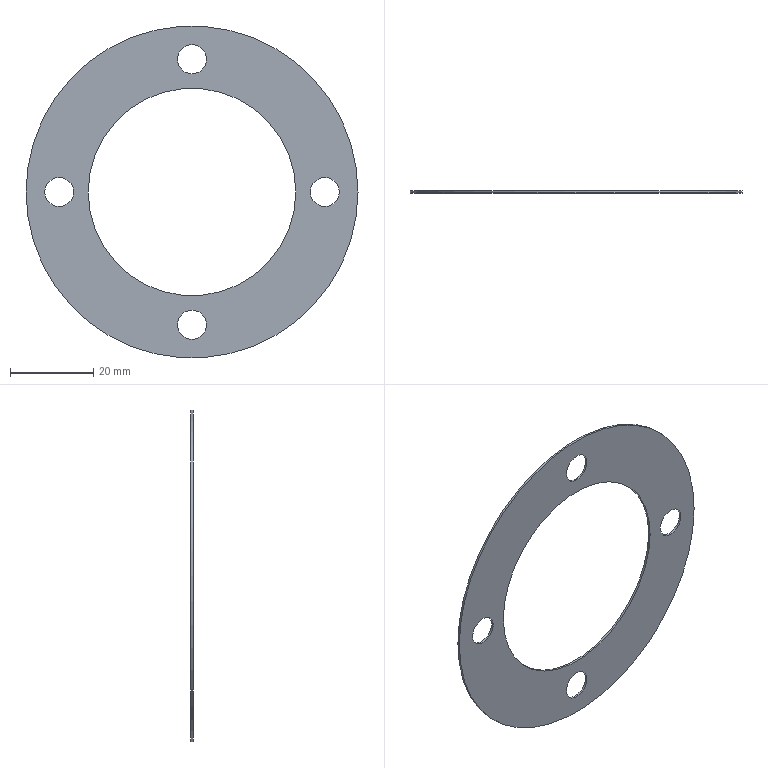Component | NX | GASKET | 1 solid | 8 faces | box 80 x 0.5 x 80 mm | volume 1455 mm3 | cylinder 6 | plane 2 | commonest cylinder face diameters 7 x4 80 x1 50 x1
STEP:
#1=CARTESIAN_POINT('',(0.,0.,0.));
#2=DIRECTION('',(0.,0.,1.));
#3=DIRECTION('',(1.,0.,0.));
#4=AXIS2_PLACEMENT_3D('',#1,#2,#3);
#5=CARTESIAN_POINT('',(40.,79.5,43.));
#6=VERTEX_POINT('',#5);
#7=CARTESIAN_POINT('',(-0.,79.5,43.));
#8=DIRECTION('',(0.,-1.,0.));
#9=DIRECTION('',(1.,0.,0.));
#10=AXIS2_PLACEMENT_3D('',#7,#8,#9);
#11=CIRCLE('',#10,40.);
#12=CARTESIAN_POINT('',(-0.,79.5,43.));
#13=DIRECTION('',(0.,1.,0.));
#14=DIRECTION('',(0.,0.,1.));
#15=AXIS2_PLACEMENT_3D('',#12,#13,#14);
#16=CYLINDRICAL_SURFACE('',#15,40.);
#17=CARTESIAN_POINT('',(7.854,0.));
#18=DIRECTION('',(-1.,0.));
#19=VECTOR('',#18,1.);
#20=LINE('',#17,#19);
#21=(GEOMETRIC_REPRESENTATION_CONTEXT(2)PARAMETRIC_REPRESENTATION_CONTEXT()REPRESENTATION_CONTEXT('',''));
#22=DEFINITIONAL_REPRESENTATION('',(#20),#21);
#23=PCURVE('',#16,#22);
#24=CARTESIAN_POINT('',(-0.,79.5,43.));
#25=DIRECTION('',(0.,-1.,0.));
#26=DIRECTION('',(0.,0.,-1.));
#27=AXIS2_PLACEMENT_3D('',#24,#25,#26);
#28=PLANE('',#27);
#29=CARTESIAN_POINT('',(0.,0.));
#30=DIRECTION('',(0.,1.));
#31=AXIS2_PLACEMENT_2D('',#29,#30);
#32=CIRCLE('',#31,40.);
#33=(GEOMETRIC_REPRESENTATION_CONTEXT(2)PARAMETRIC_REPRESENTATION_CONTEXT()REPRESENTATION_CONTEXT('',''));
#34=DEFINITIONAL_REPRESENTATION('',(#32),#33);
#35=PCURVE('',#28,#34);
#36=SURFACE_CURVE('',#11,(#23,#35),.PCURVE_S1.);
#37=EDGE_CURVE('',#6,#6,#36,.T.);
#38=ORIENTED_EDGE('',*,*,#37,.F.);
#39=CARTESIAN_POINT('',(40.,80.,43.));
#40=VERTEX_POINT('',#39);
#41=CARTESIAN_POINT('',(40.,79.5,43.));
#42=CARTESIAN_POINT('',(40.,80.,43.));
#43=B_SPLINE_CURVE_WITH_KNOTS('',1,(#41,#42),.UNSPECIFIED.,.F.,.F.,(2,2),(0.,0.5),.PIECEWISE_BEZIER_KNOTS.);
#44=CARTESIAN_POINT('',(7.854,0.));
#45=DIRECTION('',(0.,1.));
#46=VECTOR('',#45,1.);
#47=LINE('',#44,#46);
#48=(GEOMETRIC_REPRESENTATION_CONTEXT(2)PARAMETRIC_REPRESENTATION_CONTEXT()REPRESENTATION_CONTEXT('',''));
#49=DEFINITIONAL_REPRESENTATION('',(#47),#48);
#50=PCURVE('',#16,#49);
#51=CARTESIAN_POINT('',(1.571,0.));
#52=DIRECTION('',(0.,1.));
#53=VECTOR('',#52,1.);
#54=LINE('',#51,#53);
#55=(GEOMETRIC_REPRESENTATION_CONTEXT(2)PARAMETRIC_REPRESENTATION_CONTEXT()REPRESENTATION_CONTEXT('',''));
#56=DEFINITIONAL_REPRESENTATION('',(#54),#55);
#57=PCURVE('',#16,#56);
#58=SEAM_CURVE('',#43,(#50,#57),.PCURVE_S1.);
#59=EDGE_CURVE('',#6,#40,#58,.T.);
#60=ORIENTED_EDGE('',*,*,#59,.T.);
#61=CARTESIAN_POINT('',(-0.,80.,43.));
#62=DIRECTION('',(0.,-1.,0.));
#63=DIRECTION('',(1.,0.,0.));
#64=AXIS2_PLACEMENT_3D('',#61,#62,#63);
#65=CIRCLE('',#64,40.);
#66=CARTESIAN_POINT('',(7.854,0.5));
#67=DIRECTION('',(-1.,0.));
#68=VECTOR('',#67,1.);
#69=LINE('',#66,#68);
#70=(GEOMETRIC_REPRESENTATION_CONTEXT(2)PARAMETRIC_REPRESENTATION_CONTEXT()REPRESENTATION_CONTEXT('',''));
#71=DEFINITIONAL_REPRESENTATION('',(#69),#70);
#72=PCURVE('',#16,#71);
#73=CARTESIAN_POINT('',(-0.,80.,43.));
#74=DIRECTION('',(0.,-1.,0.));
#75=DIRECTION('',(0.,0.,-1.));
#76=AXIS2_PLACEMENT_3D('',#73,#74,#75);
#77=PLANE('',#76);
#78=CARTESIAN_POINT('',(0.,0.));
#79=DIRECTION('',(0.,1.));
#80=AXIS2_PLACEMENT_2D('',#78,#79);
#81=CIRCLE('',#80,40.);
#82=(GEOMETRIC_REPRESENTATION_CONTEXT(2)PARAMETRIC_REPRESENTATION_CONTEXT()REPRESENTATION_CONTEXT('',''));
#83=DEFINITIONAL_REPRESENTATION('',(#81),#82);
#84=PCURVE('',#77,#83);
#85=SURFACE_CURVE('',#65,(#72,#84),.PCURVE_S1.);
#86=EDGE_CURVE('',#40,#40,#85,.T.);
#87=ORIENTED_EDGE('',*,*,#86,.T.);
#88=ORIENTED_EDGE('',*,*,#59,.F.);
#89=EDGE_LOOP('',(#38,#60,#87,#88));
#90=FACE_BOUND('',#89,.T.);
#91=ADVANCED_FACE('',(#90),#16,.T.);
#92=CARTESIAN_POINT('',(25.,79.5,43.));
#93=VERTEX_POINT('',#92);
#94=CARTESIAN_POINT('',(-0.,79.5,43.));
#95=DIRECTION('',(0.,-1.,0.));
#96=DIRECTION('',(1.,0.,0.));
#97=AXIS2_PLACEMENT_3D('',#94,#95,#96);
#98=CIRCLE('',#97,25.);
#99=CARTESIAN_POINT('',(-0.,79.5,43.));
#100=DIRECTION('',(0.,1.,0.));
#101=DIRECTION('',(0.,0.,1.));
#102=AXIS2_PLACEMENT_3D('',#99,#100,#101);
#103=CYLINDRICAL_SURFACE('',#102,25.);
#104=CARTESIAN_POINT('',(7.854,0.));
#105=DIRECTION('',(-1.,0.));
#106=VECTOR('',#105,1.);
#107=LINE('',#104,#106);
#108=(GEOMETRIC_REPRESENTATION_CONTEXT(2)PARAMETRIC_REPRESENTATION_CONTEXT()REPRESENTATION_CONTEXT('',''));
#109=DEFINITIONAL_REPRESENTATION('',(#107),#108);
#110=PCURVE('',#103,#109);
#111=CARTESIAN_POINT('',(0.,0.));
#112=DIRECTION('',(0.,1.));
#113=AXIS2_PLACEMENT_2D('',#111,#112);
#114=CIRCLE('',#113,25.);
#115=(GEOMETRIC_REPRESENTATION_CONTEXT(2)PARAMETRIC_REPRESENTATION_CONTEXT()REPRESENTATION_CONTEXT('',''));
#116=DEFINITIONAL_REPRESENTATION('',(#114),#115);
#117=PCURVE('',#28,#116);
#118=SURFACE_CURVE('',#98,(#110,#117),.PCURVE_S1.);
#119=EDGE_CURVE('',#93,#93,#118,.T.);
#120=ORIENTED_EDGE('',*,*,#119,.F.);
#121=CARTESIAN_POINT('',(25.,80.,43.));
#122=VERTEX_POINT('',#121);
#123=CARTESIAN_POINT('',(25.,79.5,43.));
#124=CARTESIAN_POINT('',(25.,80.,43.));
#125=B_SPLINE_CURVE_WITH_KNOTS('',1,(#123,#124),.UNSPECIFIED.,.F.,.F.,(2,2),(0.,0.5),.PIECEWISE_BEZIER_KNOTS.);
#126=CARTESIAN_POINT('',(7.854,0.));
#127=DIRECTION('',(0.,1.));
#128=VECTOR('',#127,1.);
#129=LINE('',#126,#128);
#130=(GEOMETRIC_REPRESENTATION_CONTEXT(2)PARAMETRIC_REPRESENTATION_CONTEXT()REPRESENTATION_CONTEXT('',''));
#131=DEFINITIONAL_REPRESENTATION('',(#129),#130);
#132=PCURVE('',#103,#131);
#133=CARTESIAN_POINT('',(1.571,0.));
#134=DIRECTION('',(0.,1.));
#135=VECTOR('',#134,1.);
#136=LINE('',#133,#135);
#137=(GEOMETRIC_REPRESENTATION_CONTEXT(2)PARAMETRIC_REPRESENTATION_CONTEXT()REPRESENTATION_CONTEXT('',''));
#138=DEFINITIONAL_REPRESENTATION('',(#136),#137);
#139=PCURVE('',#103,#138);
#140=SEAM_CURVE('',#125,(#132,#139),.PCURVE_S1.);
#141=EDGE_CURVE('',#93,#122,#140,.T.);
#142=ORIENTED_EDGE('',*,*,#141,.T.);
#143=CARTESIAN_POINT('',(-0.,80.,43.));
#144=DIRECTION('',(0.,-1.,0.));
#145=DIRECTION('',(1.,0.,0.));
#146=AXIS2_PLACEMENT_3D('',#143,#144,#145);
#147=CIRCLE('',#146,25.);
#148=CARTESIAN_POINT('',(7.854,0.5));
#149=DIRECTION('',(-1.,0.));
#150=VECTOR('',#149,1.);
#151=LINE('',#148,#150);
#152=(GEOMETRIC_REPRESENTATION_CONTEXT(2)PARAMETRIC_REPRESENTATION_CONTEXT()REPRESENTATION_CONTEXT('',''));
#153=DEFINITIONAL_REPRESENTATION('',(#151),#152);
#154=PCURVE('',#103,#153);
#155=CARTESIAN_POINT('',(0.,0.));
#156=DIRECTION('',(0.,1.));
#157=AXIS2_PLACEMENT_2D('',#155,#156);
#158=CIRCLE('',#157,25.);
#159=(GEOMETRIC_REPRESENTATION_CONTEXT(2)PARAMETRIC_REPRESENTATION_CONTEXT()REPRESENTATION_CONTEXT('',''));
#160=DEFINITIONAL_REPRESENTATION('',(#158),#159);
#161=PCURVE('',#77,#160);
#162=SURFACE_CURVE('',#147,(#154,#161),.PCURVE_S1.);
#163=EDGE_CURVE('',#122,#122,#162,.T.);
#164=ORIENTED_EDGE('',*,*,#163,.T.);
#165=ORIENTED_EDGE('',*,*,#141,.F.);
#166=EDGE_LOOP('',(#120,#142,#164,#165));
#167=FACE_BOUND('',#166,.F.);
#168=ADVANCED_FACE('',(#167),#103,.F.);
#169=CARTESIAN_POINT('',(32.,79.5,46.5));
#170=VERTEX_POINT('',#169);
#171=CARTESIAN_POINT('',(32.,79.5,43.));
#172=DIRECTION('',(0.,1.,0.));
#173=DIRECTION('',(0.,0.,1.));
#174=AXIS2_PLACEMENT_3D('',#171,#172,#173);
#175=CIRCLE('',#174,3.5);
#176=CARTESIAN_POINT('',(-3.5,32.));
#177=CARTESIAN_POINT('',(-3.5,38.062));
#178=CARTESIAN_POINT('',(1.75,35.031));
#179=CARTESIAN_POINT('',(7.,32.));
#180=CARTESIAN_POINT('',(1.75,28.969));
#181=CARTESIAN_POINT('',(-3.5,25.938));
#182=CARTESIAN_POINT('',(-3.5,32.));
#183=(BOUNDED_CURVE()B_SPLINE_CURVE(2,(#176,#177,#178,#179,#180,#181,#182),.UNSPECIFIED.,.T.,.F.)B_SPLINE_CURVE_WITH_KNOTS((1,2,2,2,2,1),(-2.094,0.,2.094,4.189,6.283,8.378),.UNSPECIFIED.)CURVE()GEOMETRIC_REPRESENTATION_ITEM()RATIONAL_B_SPLINE_CURVE((1.,0.5,1.,0.5,1.,0.5,1.))REPRESENTATION_ITEM(''));
#184=(GEOMETRIC_REPRESENTATION_CONTEXT(2)PARAMETRIC_REPRESENTATION_CONTEXT()REPRESENTATION_CONTEXT('',''));
#185=DEFINITIONAL_REPRESENTATION('',(#183),#184);
#186=PCURVE('',#28,#185);
#187=CARTESIAN_POINT('',(32.,79.5,43.));
#188=DIRECTION('',(0.,1.,0.));
#189=DIRECTION('',(0.,0.,1.));
#190=AXIS2_PLACEMENT_3D('',#187,#188,#189);
#191=CYLINDRICAL_SURFACE('',#190,3.5);
#192=CARTESIAN_POINT('',(0.,0.));
#193=DIRECTION('',(1.,0.));
#194=VECTOR('',#193,1.);
#195=LINE('',#192,#194);
#196=(GEOMETRIC_REPRESENTATION_CONTEXT(2)PARAMETRIC_REPRESENTATION_CONTEXT()REPRESENTATION_CONTEXT('',''));
#197=DEFINITIONAL_REPRESENTATION('',(#195),#196);
#198=PCURVE('',#191,#197);
#199=SURFACE_CURVE('',#175,(#186,#198),.PCURVE_S1.);
#200=EDGE_CURVE('',#170,#170,#199,.T.);
#201=ORIENTED_EDGE('',*,*,#200,.T.);
#202=EDGE_LOOP('',(#201));
#203=FACE_BOUND('',#202,.T.);
#204=CARTESIAN_POINT('',(0.,79.5,78.5));
#205=VERTEX_POINT('',#204);
#206=CARTESIAN_POINT('',(0.,79.5,75.));
#207=DIRECTION('',(0.,1.,0.));
#208=DIRECTION('',(0.,0.,1.));
#209=AXIS2_PLACEMENT_3D('',#206,#207,#208);
#210=CIRCLE('',#209,3.5);
#211=CARTESIAN_POINT('',(-35.5,0.));
#212=CARTESIAN_POINT('',(-35.5,6.062));
#213=CARTESIAN_POINT('',(-30.25,3.031));
#214=CARTESIAN_POINT('',(-25.,0.));
#215=CARTESIAN_POINT('',(-30.25,-3.031));
#216=CARTESIAN_POINT('',(-35.5,-6.062));
#217=CARTESIAN_POINT('',(-35.5,0.));
#218=(BOUNDED_CURVE()B_SPLINE_CURVE(2,(#211,#212,#213,#214,#215,#216,#217),.UNSPECIFIED.,.T.,.F.)B_SPLINE_CURVE_WITH_KNOTS((1,2,2,2,2,1),(-2.094,0.,2.094,4.189,6.283,8.378),.UNSPECIFIED.)CURVE()GEOMETRIC_REPRESENTATION_ITEM()RATIONAL_B_SPLINE_CURVE((1.,0.5,1.,0.5,1.,0.5,1.))REPRESENTATION_ITEM(''));
#219=(GEOMETRIC_REPRESENTATION_CONTEXT(2)PARAMETRIC_REPRESENTATION_CONTEXT()REPRESENTATION_CONTEXT('',''));
#220=DEFINITIONAL_REPRESENTATION('',(#218),#219);
#221=PCURVE('',#28,#220);
#222=CARTESIAN_POINT('',(0.,79.5,75.));
#223=DIRECTION('',(0.,1.,0.));
#224=DIRECTION('',(0.,0.,1.));
#225=AXIS2_PLACEMENT_3D('',#222,#223,#224);
#226=CYLINDRICAL_SURFACE('',#225,3.5);
#227=CARTESIAN_POINT('',(0.,0.));
#228=DIRECTION('',(1.,0.));
#229=VECTOR('',#228,1.);
#230=LINE('',#227,#229);
#231=(GEOMETRIC_REPRESENTATION_CONTEXT(2)PARAMETRIC_REPRESENTATION_CONTEXT()REPRESENTATION_CONTEXT('',''));
#232=DEFINITIONAL_REPRESENTATION('',(#230),#231);
#233=PCURVE('',#226,#232);
#234=SURFACE_CURVE('',#210,(#221,#233),.PCURVE_S1.);
#235=EDGE_CURVE('',#205,#205,#234,.T.);
#236=ORIENTED_EDGE('',*,*,#235,.T.);
#237=EDGE_LOOP('',(#236));
#238=FACE_BOUND('',#237,.T.);
#239=CARTESIAN_POINT('',(-0.,79.5,14.5));
#240=VERTEX_POINT('',#239);
#241=CARTESIAN_POINT('',(-0.,79.5,11.));
#242=DIRECTION('',(0.,1.,0.));
#243=DIRECTION('',(0.,0.,1.));
#244=AXIS2_PLACEMENT_3D('',#241,#242,#243);
#245=CIRCLE('',#244,3.5);
#246=CARTESIAN_POINT('',(28.5,-0.));
#247=CARTESIAN_POINT('',(28.5,6.062));
#248=CARTESIAN_POINT('',(33.75,3.031));
#249=CARTESIAN_POINT('',(39.,-0.));
#250=CARTESIAN_POINT('',(33.75,-3.031));
#251=CARTESIAN_POINT('',(28.5,-6.062));
#252=CARTESIAN_POINT('',(28.5,-0.));
#253=(BOUNDED_CURVE()B_SPLINE_CURVE(2,(#246,#247,#248,#249,#250,#251,#252),.UNSPECIFIED.,.T.,.F.)B_SPLINE_CURVE_WITH_KNOTS((1,2,2,2,2,1),(-2.094,0.,2.094,4.189,6.283,8.378),.UNSPECIFIED.)CURVE()GEOMETRIC_REPRESENTATION_ITEM()RATIONAL_B_SPLINE_CURVE((1.,0.5,1.,0.5,1.,0.5,1.))REPRESENTATION_ITEM(''));
#254=(GEOMETRIC_REPRESENTATION_CONTEXT(2)PARAMETRIC_REPRESENTATION_CONTEXT()REPRESENTATION_CONTEXT('',''));
#255=DEFINITIONAL_REPRESENTATION('',(#253),#254);
#256=PCURVE('',#28,#255);
#257=CARTESIAN_POINT('',(-0.,79.5,11.));
#258=DIRECTION('',(0.,1.,0.));
#259=DIRECTION('',(0.,0.,1.));
#260=AXIS2_PLACEMENT_3D('',#257,#258,#259);
#261=CYLINDRICAL_SURFACE('',#260,3.5);
#262=CARTESIAN_POINT('',(0.,0.));
#263=DIRECTION('',(1.,0.));
#264=VECTOR('',#263,1.);
#265=LINE('',#262,#264);
#266=(GEOMETRIC_REPRESENTATION_CONTEXT(2)PARAMETRIC_REPRESENTATION_CONTEXT()REPRESENTATION_CONTEXT('',''));
#267=DEFINITIONAL_REPRESENTATION('',(#265),#266);
#268=PCURVE('',#261,#267);
#269=SURFACE_CURVE('',#245,(#256,#268),.PCURVE_S1.);
#270=EDGE_CURVE('',#240,#240,#269,.T.);
#271=ORIENTED_EDGE('',*,*,#270,.T.);
#272=EDGE_LOOP('',(#271));
#273=FACE_BOUND('',#272,.T.);
#274=CARTESIAN_POINT('',(-32.,79.5,46.5));
#275=VERTEX_POINT('',#274);
#276=CARTESIAN_POINT('',(-32.,79.5,43.));
#277=DIRECTION('',(0.,1.,0.));
#278=DIRECTION('',(0.,0.,1.));
#279=AXIS2_PLACEMENT_3D('',#276,#277,#278);
#280=CIRCLE('',#279,3.5);
#281=CARTESIAN_POINT('',(-3.5,-32.));
#282=CARTESIAN_POINT('',(-3.5,-25.938));
#283=CARTESIAN_POINT('',(1.75,-28.969));
#284=CARTESIAN_POINT('',(7.,-32.));
#285=CARTESIAN_POINT('',(1.75,-35.031));
#286=CARTESIAN_POINT('',(-3.5,-38.062));
#287=CARTESIAN_POINT('',(-3.5,-32.));
#288=(BOUNDED_CURVE()B_SPLINE_CURVE(2,(#281,#282,#283,#284,#285,#286,#287),.UNSPECIFIED.,.T.,.F.)B_SPLINE_CURVE_WITH_KNOTS((1,2,2,2,2,1),(-2.094,0.,2.094,4.189,6.283,8.378),.UNSPECIFIED.)CURVE()GEOMETRIC_REPRESENTATION_ITEM()RATIONAL_B_SPLINE_CURVE((1.,0.5,1.,0.5,1.,0.5,1.))REPRESENTATION_ITEM(''));
#289=(GEOMETRIC_REPRESENTATION_CONTEXT(2)PARAMETRIC_REPRESENTATION_CONTEXT()REPRESENTATION_CONTEXT('',''));
#290=DEFINITIONAL_REPRESENTATION('',(#288),#289);
#291=PCURVE('',#28,#290);
#292=CARTESIAN_POINT('',(-32.,79.5,43.));
#293=DIRECTION('',(0.,1.,0.));
#294=DIRECTION('',(0.,0.,1.));
#295=AXIS2_PLACEMENT_3D('',#292,#293,#294);
#296=CYLINDRICAL_SURFACE('',#295,3.5);
#297=CARTESIAN_POINT('',(0.,0.));
#298=DIRECTION('',(1.,0.));
#299=VECTOR('',#298,1.);
#300=LINE('',#297,#299);
#301=(GEOMETRIC_REPRESENTATION_CONTEXT(2)PARAMETRIC_REPRESENTATION_CONTEXT()REPRESENTATION_CONTEXT('',''));
#302=DEFINITIONAL_REPRESENTATION('',(#300),#301);
#303=PCURVE('',#296,#302);
#304=SURFACE_CURVE('',#280,(#291,#303),.PCURVE_S1.);
#305=EDGE_CURVE('',#275,#275,#304,.T.);
#306=ORIENTED_EDGE('',*,*,#305,.T.);
#307=EDGE_LOOP('',(#306));
#308=FACE_BOUND('',#307,.T.);
#309=ORIENTED_EDGE('',*,*,#37,.T.);
#310=EDGE_LOOP('',(#309));
#311=FACE_BOUND('',#310,.T.);
#312=ORIENTED_EDGE('',*,*,#119,.F.);
#313=EDGE_LOOP('',(#312));
#314=FACE_BOUND('',#313,.T.);
#315=ADVANCED_FACE('',(#203,#238,#273,#308,#311,#314),#28,.T.);
#316=CARTESIAN_POINT('',(32.,80.,39.5));
#317=VERTEX_POINT('',#316);
#318=CARTESIAN_POINT('',(32.,80.,46.5));
#319=VERTEX_POINT('',#318);
#320=CARTESIAN_POINT('',(32.,80.,43.));
#321=DIRECTION('',(0.,-1.,0.));
#322=DIRECTION('',(0.,0.,-1.));
#323=AXIS2_PLACEMENT_3D('',#320,#321,#322);
#324=CIRCLE('',#323,3.5);
#325=CARTESIAN_POINT('',(0.,32.));
#326=DIRECTION('',(1.,0.));
#327=AXIS2_PLACEMENT_2D('',#325,#326);
#328=CIRCLE('',#327,3.5);
#329=(GEOMETRIC_REPRESENTATION_CONTEXT(2)PARAMETRIC_REPRESENTATION_CONTEXT()REPRESENTATION_CONTEXT('',''));
#330=DEFINITIONAL_REPRESENTATION('',(#328),#329);
#331=PCURVE('',#77,#330);
#332=CARTESIAN_POINT('',(3.142,0.5));
#333=DIRECTION('',(-1.,0.));
#334=VECTOR('',#333,1.);
#335=LINE('',#332,#334);
#336=(GEOMETRIC_REPRESENTATION_CONTEXT(2)PARAMETRIC_REPRESENTATION_CONTEXT()REPRESENTATION_CONTEXT('',''));
#337=DEFINITIONAL_REPRESENTATION('',(#335),#336);
#338=PCURVE('',#191,#337);
#339=SURFACE_CURVE('',#324,(#331,#338),.PCURVE_S1.);
#340=EDGE_CURVE('',#317,#319,#339,.T.);
#341=ORIENTED_EDGE('',*,*,#340,.T.);
#342=CARTESIAN_POINT('',(32.,80.,43.));
#343=DIRECTION('',(0.,-1.,0.));
#344=DIRECTION('',(0.,0.,-1.));
#345=AXIS2_PLACEMENT_3D('',#342,#343,#344);
#346=CIRCLE('',#345,3.5);
#347=CARTESIAN_POINT('',(0.,32.));
#348=DIRECTION('',(1.,0.));
#349=AXIS2_PLACEMENT_2D('',#347,#348);
#350=CIRCLE('',#349,3.5);
#351=(GEOMETRIC_REPRESENTATION_CONTEXT(2)PARAMETRIC_REPRESENTATION_CONTEXT()REPRESENTATION_CONTEXT('',''));
#352=DEFINITIONAL_REPRESENTATION('',(#350),#351);
#353=PCURVE('',#77,#352);
#354=CARTESIAN_POINT('',(9.425,0.5));
#355=DIRECTION('',(-1.,0.));
#356=VECTOR('',#355,1.);
#357=LINE('',#354,#356);
#358=(GEOMETRIC_REPRESENTATION_CONTEXT(2)PARAMETRIC_REPRESENTATION_CONTEXT()REPRESENTATION_CONTEXT('',''));
#359=DEFINITIONAL_REPRESENTATION('',(#357),#358);
#360=PCURVE('',#191,#359);
#361=SURFACE_CURVE('',#346,(#353,#360),.PCURVE_S1.);
#362=EDGE_CURVE('',#319,#317,#361,.T.);
#363=ORIENTED_EDGE('',*,*,#362,.T.);
#364=EDGE_LOOP('',(#341,#363));
#365=FACE_BOUND('',#364,.T.);
#366=CARTESIAN_POINT('',(0.,80.,71.5));
#367=VERTEX_POINT('',#366);
#368=CARTESIAN_POINT('',(0.,80.,78.5));
#369=VERTEX_POINT('',#368);
#370=CARTESIAN_POINT('',(0.,80.,75.));
#371=DIRECTION('',(0.,-1.,0.));
#372=DIRECTION('',(0.,0.,-1.));
#373=AXIS2_PLACEMENT_3D('',#370,#371,#372);
#374=CIRCLE('',#373,3.5);
#375=CARTESIAN_POINT('',(-32.,0.));
#376=DIRECTION('',(1.,0.));
#377=AXIS2_PLACEMENT_2D('',#375,#376);
#378=CIRCLE('',#377,3.5);
#379=(GEOMETRIC_REPRESENTATION_CONTEXT(2)PARAMETRIC_REPRESENTATION_CONTEXT()REPRESENTATION_CONTEXT('',''));
#380=DEFINITIONAL_REPRESENTATION('',(#378),#379);
#381=PCURVE('',#77,#380);
#382=CARTESIAN_POINT('',(3.142,0.5));
#383=DIRECTION('',(-1.,0.));
#384=VECTOR('',#383,1.);
#385=LINE('',#382,#384);
#386=(GEOMETRIC_REPRESENTATION_CONTEXT(2)PARAMETRIC_REPRESENTATION_CONTEXT()REPRESENTATION_CONTEXT('',''));
#387=DEFINITIONAL_REPRESENTATION('',(#385),#386);
#388=PCURVE('',#226,#387);
#389=SURFACE_CURVE('',#374,(#381,#388),.PCURVE_S1.);
#390=EDGE_CURVE('',#367,#369,#389,.T.);
#391=ORIENTED_EDGE('',*,*,#390,.T.);
#392=CARTESIAN_POINT('',(0.,80.,75.));
#393=DIRECTION('',(0.,-1.,0.));
#394=DIRECTION('',(0.,0.,-1.));
#395=AXIS2_PLACEMENT_3D('',#392,#393,#394);
#396=CIRCLE('',#395,3.5);
#397=CARTESIAN_POINT('',(-32.,0.));
#398=DIRECTION('',(1.,0.));
#399=AXIS2_PLACEMENT_2D('',#397,#398);
#400=CIRCLE('',#399,3.5);
#401=(GEOMETRIC_REPRESENTATION_CONTEXT(2)PARAMETRIC_REPRESENTATION_CONTEXT()REPRESENTATION_CONTEXT('',''));
#402=DEFINITIONAL_REPRESENTATION('',(#400),#401);
#403=PCURVE('',#77,#402);
#404=CARTESIAN_POINT('',(9.425,0.5));
#405=DIRECTION('',(-1.,0.));
#406=VECTOR('',#405,1.);
#407=LINE('',#404,#406);
#408=(GEOMETRIC_REPRESENTATION_CONTEXT(2)PARAMETRIC_REPRESENTATION_CONTEXT()REPRESENTATION_CONTEXT('',''));
#409=DEFINITIONAL_REPRESENTATION('',(#407),#408);
#410=PCURVE('',#226,#409);
#411=SURFACE_CURVE('',#396,(#403,#410),.PCURVE_S1.);
#412=EDGE_CURVE('',#369,#367,#411,.T.);
#413=ORIENTED_EDGE('',*,*,#412,.T.);
#414=EDGE_LOOP('',(#391,#413));
#415=FACE_BOUND('',#414,.T.);
#416=CARTESIAN_POINT('',(-0.,80.,7.5));
#417=VERTEX_POINT('',#416);
#418=CARTESIAN_POINT('',(-0.,80.,14.5));
#419=VERTEX_POINT('',#418);
#420=CARTESIAN_POINT('',(-0.,80.,11.));
#421=DIRECTION('',(0.,-1.,0.));
#422=DIRECTION('',(0.,0.,-1.));
#423=AXIS2_PLACEMENT_3D('',#420,#421,#422);
#424=CIRCLE('',#423,3.5);
#425=CARTESIAN_POINT('',(32.,-0.));
#426=DIRECTION('',(1.,0.));
#427=AXIS2_PLACEMENT_2D('',#425,#426);
#428=CIRCLE('',#427,3.5);
#429=(GEOMETRIC_REPRESENTATION_CONTEXT(2)PARAMETRIC_REPRESENTATION_CONTEXT()REPRESENTATION_CONTEXT('',''));
#430=DEFINITIONAL_REPRESENTATION('',(#428),#429);
#431=PCURVE('',#77,#430);
#432=CARTESIAN_POINT('',(3.142,0.5));
#433=DIRECTION('',(-1.,0.));
#434=VECTOR('',#433,1.);
#435=LINE('',#432,#434);
#436=(GEOMETRIC_REPRESENTATION_CONTEXT(2)PARAMETRIC_REPRESENTATION_CONTEXT()REPRESENTATION_CONTEXT('',''));
#437=DEFINITIONAL_REPRESENTATION('',(#435),#436);
#438=PCURVE('',#261,#437);
#439=SURFACE_CURVE('',#424,(#431,#438),.PCURVE_S1.);
#440=EDGE_CURVE('',#417,#419,#439,.T.);
#441=ORIENTED_EDGE('',*,*,#440,.T.);
#442=CARTESIAN_POINT('',(-0.,80.,11.));
#443=DIRECTION('',(0.,-1.,0.));
#444=DIRECTION('',(0.,0.,-1.));
#445=AXIS2_PLACEMENT_3D('',#442,#443,#444);
#446=CIRCLE('',#445,3.5);
#447=CARTESIAN_POINT('',(32.,-0.));
#448=DIRECTION('',(1.,0.));
#449=AXIS2_PLACEMENT_2D('',#447,#448);
#450=CIRCLE('',#449,3.5);
#451=(GEOMETRIC_REPRESENTATION_CONTEXT(2)PARAMETRIC_REPRESENTATION_CONTEXT()REPRESENTATION_CONTEXT('',''));
#452=DEFINITIONAL_REPRESENTATION('',(#450),#451);
#453=PCURVE('',#77,#452);
#454=CARTESIAN_POINT('',(9.425,0.5));
#455=DIRECTION('',(-1.,0.));
#456=VECTOR('',#455,1.);
#457=LINE('',#454,#456);
#458=(GEOMETRIC_REPRESENTATION_CONTEXT(2)PARAMETRIC_REPRESENTATION_CONTEXT()REPRESENTATION_CONTEXT('',''));
#459=DEFINITIONAL_REPRESENTATION('',(#457),#458);
#460=PCURVE('',#261,#459);
#461=SURFACE_CURVE('',#446,(#453,#460),.PCURVE_S1.);
#462=EDGE_CURVE('',#419,#417,#461,.T.);
#463=ORIENTED_EDGE('',*,*,#462,.T.);
#464=EDGE_LOOP('',(#441,#463));
#465=FACE_BOUND('',#464,.T.);
#466=CARTESIAN_POINT('',(-32.,80.,39.5));
#467=VERTEX_POINT('',#466);
#468=CARTESIAN_POINT('',(-32.,80.,46.5));
#469=VERTEX_POINT('',#468);
#470=CARTESIAN_POINT('',(-32.,80.,43.));
#471=DIRECTION('',(0.,-1.,0.));
#472=DIRECTION('',(0.,0.,-1.));
#473=AXIS2_PLACEMENT_3D('',#470,#471,#472);
#474=CIRCLE('',#473,3.5);
#475=CARTESIAN_POINT('',(0.,-32.));
#476=DIRECTION('',(1.,0.));
#477=AXIS2_PLACEMENT_2D('',#475,#476);
#478=CIRCLE('',#477,3.5);
#479=(GEOMETRIC_REPRESENTATION_CONTEXT(2)PARAMETRIC_REPRESENTATION_CONTEXT()REPRESENTATION_CONTEXT('',''));
#480=DEFINITIONAL_REPRESENTATION('',(#478),#479);
#481=PCURVE('',#77,#480);
#482=CARTESIAN_POINT('',(3.142,0.5));
#483=DIRECTION('',(-1.,0.));
#484=VECTOR('',#483,1.);
#485=LINE('',#482,#484);
#486=(GEOMETRIC_REPRESENTATION_CONTEXT(2)PARAMETRIC_REPRESENTATION_CONTEXT()REPRESENTATION_CONTEXT('',''));
#487=DEFINITIONAL_REPRESENTATION('',(#485),#486);
#488=PCURVE('',#296,#487);
#489=SURFACE_CURVE('',#474,(#481,#488),.PCURVE_S1.);
#490=EDGE_CURVE('',#467,#469,#489,.T.);
#491=ORIENTED_EDGE('',*,*,#490,.T.);
#492=CARTESIAN_POINT('',(-32.,80.,43.));
#493=DIRECTION('',(0.,-1.,0.));
#494=DIRECTION('',(0.,0.,-1.));
#495=AXIS2_PLACEMENT_3D('',#492,#493,#494);
#496=CIRCLE('',#495,3.5);
#497=CARTESIAN_POINT('',(0.,-32.));
#498=DIRECTION('',(1.,0.));
#499=AXIS2_PLACEMENT_2D('',#497,#498);
#500=CIRCLE('',#499,3.5);
#501=(GEOMETRIC_REPRESENTATION_CONTEXT(2)PARAMETRIC_REPRESENTATION_CONTEXT()REPRESENTATION_CONTEXT('',''));
#502=DEFINITIONAL_REPRESENTATION('',(#500),#501);
#503=PCURVE('',#77,#502);
#504=CARTESIAN_POINT('',(9.425,0.5));
#505=DIRECTION('',(-1.,0.));
#506=VECTOR('',#505,1.);
#507=LINE('',#504,#506);
#508=(GEOMETRIC_REPRESENTATION_CONTEXT(2)PARAMETRIC_REPRESENTATION_CONTEXT()REPRESENTATION_CONTEXT('',''));
#509=DEFINITIONAL_REPRESENTATION('',(#507),#508);
#510=PCURVE('',#296,#509);
#511=SURFACE_CURVE('',#496,(#503,#510),.PCURVE_S1.);
#512=EDGE_CURVE('',#469,#467,#511,.T.);
#513=ORIENTED_EDGE('',*,*,#512,.T.);
#514=EDGE_LOOP('',(#491,#513));
#515=FACE_BOUND('',#514,.T.);
#516=ORIENTED_EDGE('',*,*,#86,.F.);
#517=EDGE_LOOP('',(#516));
#518=FACE_BOUND('',#517,.T.);
#519=ORIENTED_EDGE('',*,*,#163,.T.);
#520=EDGE_LOOP('',(#519));
#521=FACE_BOUND('',#520,.T.);
#522=ADVANCED_FACE('',(#365,#415,#465,#515,#518,#521),#77,.F.);
#523=ORIENTED_EDGE('',*,*,#305,.T.);
#524=CARTESIAN_POINT('',(-32.,79.5,46.5));
#525=CARTESIAN_POINT('',(-32.,80.,46.5));
#526=B_SPLINE_CURVE_WITH_KNOTS('',1,(#524,#525),.UNSPECIFIED.,.F.,.F.,(2,2),(0.,0.5),.PIECEWISE_BEZIER_KNOTS.);
#527=CARTESIAN_POINT('',(6.283,0.));
#528=DIRECTION('',(0.,1.));
#529=VECTOR('',#528,1.);
#530=LINE('',#527,#529);
#531=(GEOMETRIC_REPRESENTATION_CONTEXT(2)PARAMETRIC_REPRESENTATION_CONTEXT()REPRESENTATION_CONTEXT('',''));
#532=DEFINITIONAL_REPRESENTATION('',(#530),#531);
#533=PCURVE('',#296,#532);
#534=CARTESIAN_POINT('',(0.,0.));
#535=DIRECTION('',(0.,1.));
#536=VECTOR('',#535,1.);
#537=LINE('',#534,#536);
#538=(GEOMETRIC_REPRESENTATION_CONTEXT(2)PARAMETRIC_REPRESENTATION_CONTEXT()REPRESENTATION_CONTEXT('',''));
#539=DEFINITIONAL_REPRESENTATION('',(#537),#538);
#540=PCURVE('',#296,#539);
#541=SEAM_CURVE('',#526,(#533,#540),.PCURVE_S1.);
#542=EDGE_CURVE('',#275,#469,#541,.T.);
#543=ORIENTED_EDGE('',*,*,#542,.T.);
#544=ORIENTED_EDGE('',*,*,#512,.T.);
#545=ORIENTED_EDGE('',*,*,#490,.T.);
#546=ORIENTED_EDGE('',*,*,#542,.F.);
#547=EDGE_LOOP('',(#523,#543,#544,#545,#546));
#548=FACE_BOUND('',#547,.F.);
#549=ADVANCED_FACE('',(#548),#296,.F.);
#550=ORIENTED_EDGE('',*,*,#270,.T.);
#551=CARTESIAN_POINT('',(-0.,79.5,14.5));
#552=CARTESIAN_POINT('',(-0.,80.,14.5));
#553=B_SPLINE_CURVE_WITH_KNOTS('',1,(#551,#552),.UNSPECIFIED.,.F.,.F.,(2,2),(0.,0.5),.PIECEWISE_BEZIER_KNOTS.);
#554=CARTESIAN_POINT('',(6.283,0.));
#555=DIRECTION('',(0.,1.));
#556=VECTOR('',#555,1.);
#557=LINE('',#554,#556);
#558=(GEOMETRIC_REPRESENTATION_CONTEXT(2)PARAMETRIC_REPRESENTATION_CONTEXT()REPRESENTATION_CONTEXT('',''));
#559=DEFINITIONAL_REPRESENTATION('',(#557),#558);
#560=PCURVE('',#261,#559);
#561=CARTESIAN_POINT('',(0.,0.));
#562=DIRECTION('',(0.,1.));
#563=VECTOR('',#562,1.);
#564=LINE('',#561,#563);
#565=(GEOMETRIC_REPRESENTATION_CONTEXT(2)PARAMETRIC_REPRESENTATION_CONTEXT()REPRESENTATION_CONTEXT('',''));
#566=DEFINITIONAL_REPRESENTATION('',(#564),#565);
#567=PCURVE('',#261,#566);
#568=SEAM_CURVE('',#553,(#560,#567),.PCURVE_S1.);
#569=EDGE_CURVE('',#240,#419,#568,.T.);
#570=ORIENTED_EDGE('',*,*,#569,.T.);
#571=ORIENTED_EDGE('',*,*,#462,.T.);
#572=ORIENTED_EDGE('',*,*,#440,.T.);
#573=ORIENTED_EDGE('',*,*,#569,.F.);
#574=EDGE_LOOP('',(#550,#570,#571,#572,#573));
#575=FACE_BOUND('',#574,.F.);
#576=ADVANCED_FACE('',(#575),#261,.F.);
#577=ORIENTED_EDGE('',*,*,#235,.T.);
#578=CARTESIAN_POINT('',(0.,79.5,78.5));
#579=CARTESIAN_POINT('',(0.,80.,78.5));
#580=B_SPLINE_CURVE_WITH_KNOTS('',1,(#578,#579),.UNSPECIFIED.,.F.,.F.,(2,2),(0.,0.5),.PIECEWISE_BEZIER_KNOTS.);
#581=CARTESIAN_POINT('',(6.283,0.));
#582=DIRECTION('',(0.,1.));
#583=VECTOR('',#582,1.);
#584=LINE('',#581,#583);
#585=(GEOMETRIC_REPRESENTATION_CONTEXT(2)PARAMETRIC_REPRESENTATION_CONTEXT()REPRESENTATION_CONTEXT('',''));
#586=DEFINITIONAL_REPRESENTATION('',(#584),#585);
#587=PCURVE('',#226,#586);
#588=CARTESIAN_POINT('',(0.,0.));
#589=DIRECTION('',(0.,1.));
#590=VECTOR('',#589,1.);
#591=LINE('',#588,#590);
#592=(GEOMETRIC_REPRESENTATION_CONTEXT(2)PARAMETRIC_REPRESENTATION_CONTEXT()REPRESENTATION_CONTEXT('',''));
#593=DEFINITIONAL_REPRESENTATION('',(#591),#592);
#594=PCURVE('',#226,#593);
#595=SEAM_CURVE('',#580,(#587,#594),.PCURVE_S1.);
#596=EDGE_CURVE('',#205,#369,#595,.T.);
#597=ORIENTED_EDGE('',*,*,#596,.T.);
#598=ORIENTED_EDGE('',*,*,#412,.T.);
#599=ORIENTED_EDGE('',*,*,#390,.T.);
#600=ORIENTED_EDGE('',*,*,#596,.F.);
#601=EDGE_LOOP('',(#577,#597,#598,#599,#600));
#602=FACE_BOUND('',#601,.F.);
#603=ADVANCED_FACE('',(#602),#226,.F.);
#604=ORIENTED_EDGE('',*,*,#200,.T.);
#605=CARTESIAN_POINT('',(32.,79.5,46.5));
#606=CARTESIAN_POINT('',(32.,80.,46.5));
#607=B_SPLINE_CURVE_WITH_KNOTS('',1,(#605,#606),.UNSPECIFIED.,.F.,.F.,(2,2),(0.,0.5),.PIECEWISE_BEZIER_KNOTS.);
#608=CARTESIAN_POINT('',(6.283,0.));
#609=DIRECTION('',(0.,1.));
#610=VECTOR('',#609,1.);
#611=LINE('',#608,#610);
#612=(GEOMETRIC_REPRESENTATION_CONTEXT(2)PARAMETRIC_REPRESENTATION_CONTEXT()REPRESENTATION_CONTEXT('',''));
#613=DEFINITIONAL_REPRESENTATION('',(#611),#612);
#614=PCURVE('',#191,#613);
#615=CARTESIAN_POINT('',(0.,0.));
#616=DIRECTION('',(0.,1.));
#617=VECTOR('',#616,1.);
#618=LINE('',#615,#617);
#619=(GEOMETRIC_REPRESENTATION_CONTEXT(2)PARAMETRIC_REPRESENTATION_CONTEXT()REPRESENTATION_CONTEXT('',''));
#620=DEFINITIONAL_REPRESENTATION('',(#618),#619);
#621=PCURVE('',#191,#620);
#622=SEAM_CURVE('',#607,(#614,#621),.PCURVE_S1.);
#623=EDGE_CURVE('',#170,#319,#622,.T.);
#624=ORIENTED_EDGE('',*,*,#623,.T.);
#625=ORIENTED_EDGE('',*,*,#362,.T.);
#626=ORIENTED_EDGE('',*,*,#340,.T.);
#627=ORIENTED_EDGE('',*,*,#623,.F.);
#628=EDGE_LOOP('',(#604,#624,#625,#626,#627));
#629=FACE_BOUND('',#628,.F.);
#630=ADVANCED_FACE('',(#629),#191,.F.);
#631=CLOSED_SHELL('',(#91,#168,#315,#522,#549,#576,#603,#630));
#632=MANIFOLD_SOLID_BREP('',#631);
#633=(LENGTH_UNIT()NAMED_UNIT(*)SI_UNIT(.MILLI.,.METRE.));
#634=UNCERTAINTY_MEASURE_WITH_UNIT(LENGTH_MEASURE(0.000005),#633,'','');
#635=(NAMED_UNIT(*)PLANE_ANGLE_UNIT()SI_UNIT($,.RADIAN.));
#636=(NAMED_UNIT(*)SI_UNIT($,.STERADIAN.)SOLID_ANGLE_UNIT());
#637=(GEOMETRIC_REPRESENTATION_CONTEXT(3)GLOBAL_UNCERTAINTY_ASSIGNED_CONTEXT((#634))GLOBAL_UNIT_ASSIGNED_CONTEXT((#633,#635,#636))REPRESENTATION_CONTEXT('',''));
#638=ADVANCED_BREP_SHAPE_REPRESENTATION('',(#4,#632),#637);